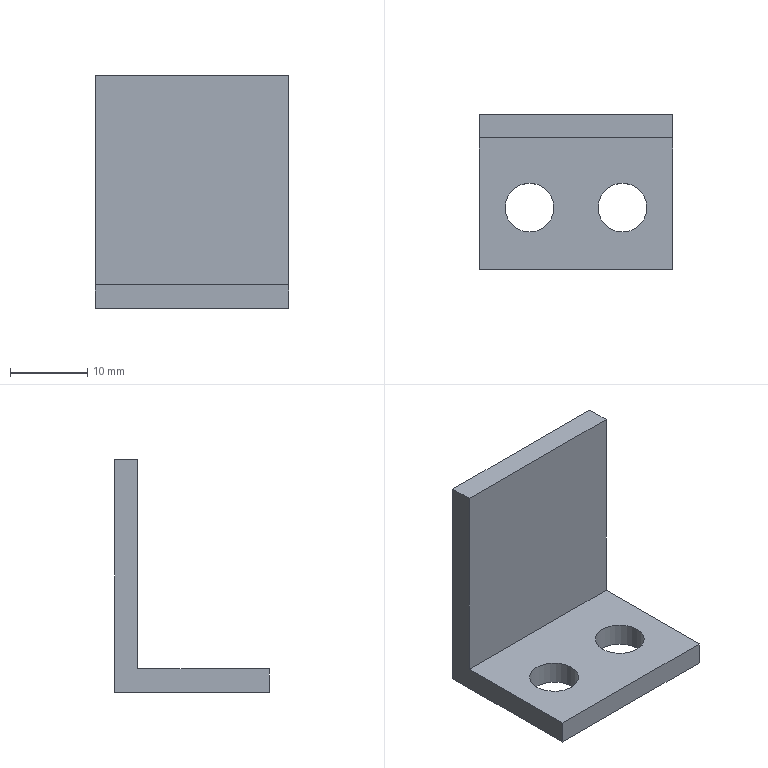Component | NX | SPRING_FIXING_PLATE | 1 solid | 10 faces | box 25 x 20 x 30 mm | volume 3338 mm3 | plane 8 | cylinder 2 | commonest cylinder face diameters 6.3 x2
STEP:
#1=CARTESIAN_POINT('',(0.,0.,0.));
#2=DIRECTION('',(0.,0.,1.));
#3=DIRECTION('',(1.,0.,0.));
#4=AXIS2_PLACEMENT_3D('',#1,#2,#3);
#5=CARTESIAN_POINT('',(-151.5,-8.,303.));
#6=VERTEX_POINT('',#5);
#7=CARTESIAN_POINT('',(-151.5,-25.,303.));
#8=VERTEX_POINT('',#7);
#9=CARTESIAN_POINT('',(-151.5,-5.,303.));
#10=DIRECTION('',(-0.,-1.,0.));
#11=VECTOR('',#10,1.);
#12=LINE('',#9,#11);
#13=CARTESIAN_POINT('',(-151.5,-5.,330.));
#14=DIRECTION('',(1.,-0.,0.));
#15=DIRECTION('',(0.,1.,0.));
#16=AXIS2_PLACEMENT_3D('',#13,#14,#15);
#17=PLANE('',#16);
#18=CARTESIAN_POINT('',(0.,-27.));
#19=DIRECTION('',(-1.,0.));
#20=VECTOR('',#19,1.);
#21=LINE('',#18,#20);
#22=(GEOMETRIC_REPRESENTATION_CONTEXT(2)PARAMETRIC_REPRESENTATION_CONTEXT()REPRESENTATION_CONTEXT('',''));
#23=DEFINITIONAL_REPRESENTATION('',(#21),#22);
#24=PCURVE('',#17,#23);
#25=CARTESIAN_POINT('',(-139.,-5.,303.));
#26=DIRECTION('',(0.,0.,1.));
#27=DIRECTION('',(1.,0.,0.));
#28=AXIS2_PLACEMENT_3D('',#25,#26,#27);
#29=PLANE('',#28);
#30=CARTESIAN_POINT('',(-12.5,0.));
#31=DIRECTION('',(-0.,-1.));
#32=VECTOR('',#31,1.);
#33=LINE('',#30,#32);
#34=(GEOMETRIC_REPRESENTATION_CONTEXT(2)PARAMETRIC_REPRESENTATION_CONTEXT()REPRESENTATION_CONTEXT('',''));
#35=DEFINITIONAL_REPRESENTATION('',(#33),#34);
#36=PCURVE('',#29,#35);
#37=SURFACE_CURVE('',#12,(#24,#36),.PCURVE_S1.);
#38=EDGE_CURVE('',#6,#8,#37,.T.);
#39=ORIENTED_EDGE('',*,*,#38,.F.);
#40=CARTESIAN_POINT('',(-151.5,-8.,330.));
#41=VERTEX_POINT('',#40);
#42=CARTESIAN_POINT('',(-151.5,-8.,330.));
#43=DIRECTION('',(0.,0.,-1.));
#44=VECTOR('',#43,1.);
#45=LINE('',#42,#44);
#46=CARTESIAN_POINT('',(-3.,0.));
#47=DIRECTION('',(0.,-1.));
#48=VECTOR('',#47,1.);
#49=LINE('',#46,#48);
#50=(GEOMETRIC_REPRESENTATION_CONTEXT(2)PARAMETRIC_REPRESENTATION_CONTEXT()REPRESENTATION_CONTEXT('',''));
#51=DEFINITIONAL_REPRESENTATION('',(#49),#50);
#52=PCURVE('',#17,#51);
#53=CARTESIAN_POINT('',(-126.5,-8.,330.));
#54=DIRECTION('',(0.,-1.,0.));
#55=DIRECTION('',(0.,0.,-1.));
#56=AXIS2_PLACEMENT_3D('',#53,#54,#55);
#57=PLANE('',#56);
#58=CARTESIAN_POINT('',(0.,-25.));
#59=DIRECTION('',(1.,0.));
#60=VECTOR('',#59,1.);
#61=LINE('',#58,#60);
#62=(GEOMETRIC_REPRESENTATION_CONTEXT(2)PARAMETRIC_REPRESENTATION_CONTEXT()REPRESENTATION_CONTEXT('',''));
#63=DEFINITIONAL_REPRESENTATION('',(#61),#62);
#64=PCURVE('',#57,#63);
#65=SURFACE_CURVE('',#45,(#52,#64),.PCURVE_S1.);
#66=EDGE_CURVE('',#41,#6,#65,.T.);
#67=ORIENTED_EDGE('',*,*,#66,.F.);
#68=CARTESIAN_POINT('',(-151.5,-5.,330.));
#69=VERTEX_POINT('',#68);
#70=CARTESIAN_POINT('',(-151.5,-5.,330.));
#71=DIRECTION('',(-0.,-1.,0.));
#72=VECTOR('',#71,1.);
#73=LINE('',#70,#72);
#74=CARTESIAN_POINT('',(0.,0.));
#75=DIRECTION('',(-1.,0.));
#76=VECTOR('',#75,1.);
#77=LINE('',#74,#76);
#78=(GEOMETRIC_REPRESENTATION_CONTEXT(2)PARAMETRIC_REPRESENTATION_CONTEXT()REPRESENTATION_CONTEXT('',''));
#79=DEFINITIONAL_REPRESENTATION('',(#77),#78);
#80=PCURVE('',#17,#79);
#81=CARTESIAN_POINT('',(-139.,-5.,330.));
#82=DIRECTION('',(0.,0.,1.));
#83=DIRECTION('',(1.,0.,0.));
#84=AXIS2_PLACEMENT_3D('',#81,#82,#83);
#85=PLANE('',#84);
#86=CARTESIAN_POINT('',(-12.5,0.));
#87=DIRECTION('',(-0.,-1.));
#88=VECTOR('',#87,1.);
#89=LINE('',#86,#88);
#90=(GEOMETRIC_REPRESENTATION_CONTEXT(2)PARAMETRIC_REPRESENTATION_CONTEXT()REPRESENTATION_CONTEXT('',''));
#91=DEFINITIONAL_REPRESENTATION('',(#89),#90);
#92=PCURVE('',#85,#91);
#93=SURFACE_CURVE('',#73,(#80,#92),.PCURVE_S1.);
#94=EDGE_CURVE('',#69,#41,#93,.T.);
#95=ORIENTED_EDGE('',*,*,#94,.F.);
#96=CARTESIAN_POINT('',(-151.5,-5.,300.));
#97=VERTEX_POINT('',#96);
#98=CARTESIAN_POINT('',(-151.5,-5.,330.));
#99=DIRECTION('',(0.,0.,-1.));
#100=VECTOR('',#99,1.);
#101=LINE('',#98,#100);
#102=CARTESIAN_POINT('',(0.,0.));
#103=DIRECTION('',(0.,-1.));
#104=VECTOR('',#103,1.);
#105=LINE('',#102,#104);
#106=(GEOMETRIC_REPRESENTATION_CONTEXT(2)PARAMETRIC_REPRESENTATION_CONTEXT()REPRESENTATION_CONTEXT('',''));
#107=DEFINITIONAL_REPRESENTATION('',(#105),#106);
#108=PCURVE('',#17,#107);
#109=CARTESIAN_POINT('',(-126.5,-5.,330.));
#110=DIRECTION('',(0.,-1.,0.));
#111=DIRECTION('',(0.,0.,-1.));
#112=AXIS2_PLACEMENT_3D('',#109,#110,#111);
#113=PLANE('',#112);
#114=CARTESIAN_POINT('',(0.,-25.));
#115=DIRECTION('',(1.,0.));
#116=VECTOR('',#115,1.);
#117=LINE('',#114,#116);
#118=(GEOMETRIC_REPRESENTATION_CONTEXT(2)PARAMETRIC_REPRESENTATION_CONTEXT()REPRESENTATION_CONTEXT('',''));
#119=DEFINITIONAL_REPRESENTATION('',(#117),#118);
#120=PCURVE('',#113,#119);
#121=SURFACE_CURVE('',#101,(#108,#120),.PCURVE_S1.);
#122=EDGE_CURVE('',#69,#97,#121,.T.);
#123=ORIENTED_EDGE('',*,*,#122,.T.);
#124=CARTESIAN_POINT('',(-151.5,-25.,300.));
#125=VERTEX_POINT('',#124);
#126=CARTESIAN_POINT('',(-151.5,-5.,300.));
#127=DIRECTION('',(-0.,-1.,0.));
#128=VECTOR('',#127,1.);
#129=LINE('',#126,#128);
#130=CARTESIAN_POINT('',(0.,-30.));
#131=DIRECTION('',(-1.,0.));
#132=VECTOR('',#131,1.);
#133=LINE('',#130,#132);
#134=(GEOMETRIC_REPRESENTATION_CONTEXT(2)PARAMETRIC_REPRESENTATION_CONTEXT()REPRESENTATION_CONTEXT('',''));
#135=DEFINITIONAL_REPRESENTATION('',(#133),#134);
#136=PCURVE('',#17,#135);
#137=CARTESIAN_POINT('',(-139.,-5.,300.));
#138=DIRECTION('',(0.,0.,1.));
#139=DIRECTION('',(1.,0.,0.));
#140=AXIS2_PLACEMENT_3D('',#137,#138,#139);
#141=PLANE('',#140);
#142=CARTESIAN_POINT('',(-12.5,0.));
#143=DIRECTION('',(-0.,-1.));
#144=VECTOR('',#143,1.);
#145=LINE('',#142,#144);
#146=(GEOMETRIC_REPRESENTATION_CONTEXT(2)PARAMETRIC_REPRESENTATION_CONTEXT()REPRESENTATION_CONTEXT('',''));
#147=DEFINITIONAL_REPRESENTATION('',(#145),#146);
#148=PCURVE('',#141,#147);
#149=SURFACE_CURVE('',#129,(#136,#148),.PCURVE_S1.);
#150=EDGE_CURVE('',#97,#125,#149,.T.);
#151=ORIENTED_EDGE('',*,*,#150,.T.);
#152=CARTESIAN_POINT('',(-151.5,-25.,330.));
#153=DIRECTION('',(0.,0.,-1.));
#154=VECTOR('',#153,1.);
#155=LINE('',#152,#154);
#156=CARTESIAN_POINT('',(-20.,0.));
#157=DIRECTION('',(0.,-1.));
#158=VECTOR('',#157,1.);
#159=LINE('',#156,#158);
#160=(GEOMETRIC_REPRESENTATION_CONTEXT(2)PARAMETRIC_REPRESENTATION_CONTEXT()REPRESENTATION_CONTEXT('',''));
#161=DEFINITIONAL_REPRESENTATION('',(#159),#160);
#162=PCURVE('',#17,#161);
#163=CARTESIAN_POINT('',(-151.5,-25.,330.));
#164=DIRECTION('',(0.,1.,0.));
#165=DIRECTION('',(0.,0.,1.));
#166=AXIS2_PLACEMENT_3D('',#163,#164,#165);
#167=PLANE('',#166);
#168=CARTESIAN_POINT('',(0.,0.));
#169=DIRECTION('',(-1.,0.));
#170=VECTOR('',#169,1.);
#171=LINE('',#168,#170);
#172=(GEOMETRIC_REPRESENTATION_CONTEXT(2)PARAMETRIC_REPRESENTATION_CONTEXT()REPRESENTATION_CONTEXT('',''));
#173=DEFINITIONAL_REPRESENTATION('',(#171),#172);
#174=PCURVE('',#167,#173);
#175=SURFACE_CURVE('',#155,(#162,#174),.PCURVE_S1.);
#176=EDGE_CURVE('',#8,#125,#175,.T.);
#177=ORIENTED_EDGE('',*,*,#176,.F.);
#178=EDGE_LOOP('',(#39,#67,#95,#123,#151,#177));
#179=FACE_BOUND('',#178,.T.);
#180=ADVANCED_FACE('',(#179),#17,.F.);
#181=CARTESIAN_POINT('',(-126.5,-25.,303.));
#182=VERTEX_POINT('',#181);
#183=CARTESIAN_POINT('',(-151.5,-25.,303.));
#184=DIRECTION('',(1.,0.,0.));
#185=VECTOR('',#184,1.);
#186=LINE('',#183,#185);
#187=CARTESIAN_POINT('',(-27.,0.));
#188=DIRECTION('',(0.,1.));
#189=VECTOR('',#188,1.);
#190=LINE('',#187,#189);
#191=(GEOMETRIC_REPRESENTATION_CONTEXT(2)PARAMETRIC_REPRESENTATION_CONTEXT()REPRESENTATION_CONTEXT('',''));
#192=DEFINITIONAL_REPRESENTATION('',(#190),#191);
#193=PCURVE('',#167,#192);
#194=CARTESIAN_POINT('',(-12.5,-20.));
#195=DIRECTION('',(1.,0.));
#196=VECTOR('',#195,1.);
#197=LINE('',#194,#196);
#198=(GEOMETRIC_REPRESENTATION_CONTEXT(2)PARAMETRIC_REPRESENTATION_CONTEXT()REPRESENTATION_CONTEXT('',''));
#199=DEFINITIONAL_REPRESENTATION('',(#197),#198);
#200=PCURVE('',#29,#199);
#201=SURFACE_CURVE('',#186,(#193,#200),.PCURVE_S1.);
#202=EDGE_CURVE('',#8,#182,#201,.T.);
#203=ORIENTED_EDGE('',*,*,#202,.F.);
#204=ORIENTED_EDGE('',*,*,#176,.T.);
#205=CARTESIAN_POINT('',(-126.5,-25.,300.));
#206=VERTEX_POINT('',#205);
#207=CARTESIAN_POINT('',(-151.5,-25.,300.));
#208=DIRECTION('',(1.,0.,0.));
#209=VECTOR('',#208,1.);
#210=LINE('',#207,#209);
#211=CARTESIAN_POINT('',(-30.,0.));
#212=DIRECTION('',(0.,1.));
#213=VECTOR('',#212,1.);
#214=LINE('',#211,#213);
#215=(GEOMETRIC_REPRESENTATION_CONTEXT(2)PARAMETRIC_REPRESENTATION_CONTEXT()REPRESENTATION_CONTEXT('',''));
#216=DEFINITIONAL_REPRESENTATION('',(#214),#215);
#217=PCURVE('',#167,#216);
#218=CARTESIAN_POINT('',(-12.5,-20.));
#219=DIRECTION('',(1.,0.));
#220=VECTOR('',#219,1.);
#221=LINE('',#218,#220);
#222=(GEOMETRIC_REPRESENTATION_CONTEXT(2)PARAMETRIC_REPRESENTATION_CONTEXT()REPRESENTATION_CONTEXT('',''));
#223=DEFINITIONAL_REPRESENTATION('',(#221),#222);
#224=PCURVE('',#141,#223);
#225=SURFACE_CURVE('',#210,(#217,#224),.PCURVE_S1.);
#226=EDGE_CURVE('',#125,#206,#225,.T.);
#227=ORIENTED_EDGE('',*,*,#226,.T.);
#228=CARTESIAN_POINT('',(-126.5,-25.,330.));
#229=DIRECTION('',(0.,0.,-1.));
#230=VECTOR('',#229,1.);
#231=LINE('',#228,#230);
#232=CARTESIAN_POINT('',(0.,25.));
#233=DIRECTION('',(-1.,0.));
#234=VECTOR('',#233,1.);
#235=LINE('',#232,#234);
#236=(GEOMETRIC_REPRESENTATION_CONTEXT(2)PARAMETRIC_REPRESENTATION_CONTEXT()REPRESENTATION_CONTEXT('',''));
#237=DEFINITIONAL_REPRESENTATION('',(#235),#236);
#238=PCURVE('',#167,#237);
#239=CARTESIAN_POINT('',(-126.5,-25.,330.));
#240=DIRECTION('',(-1.,-0.,0.));
#241=DIRECTION('',(0.,-1.,0.));
#242=AXIS2_PLACEMENT_3D('',#239,#240,#241);
#243=PLANE('',#242);
#244=CARTESIAN_POINT('',(0.,0.));
#245=DIRECTION('',(0.,-1.));
#246=VECTOR('',#245,1.);
#247=LINE('',#244,#246);
#248=(GEOMETRIC_REPRESENTATION_CONTEXT(2)PARAMETRIC_REPRESENTATION_CONTEXT()REPRESENTATION_CONTEXT('',''));
#249=DEFINITIONAL_REPRESENTATION('',(#247),#248);
#250=PCURVE('',#243,#249);
#251=SURFACE_CURVE('',#231,(#238,#250),.PCURVE_S1.);
#252=EDGE_CURVE('',#182,#206,#251,.T.);
#253=ORIENTED_EDGE('',*,*,#252,.F.);
#254=EDGE_LOOP('',(#203,#204,#227,#253));
#255=FACE_BOUND('',#254,.T.);
#256=ADVANCED_FACE('',(#255),#167,.F.);
#257=CARTESIAN_POINT('',(-126.5,-8.,303.));
#258=VERTEX_POINT('',#257);
#259=CARTESIAN_POINT('',(-126.5,-25.,303.));
#260=DIRECTION('',(-0.,1.,0.));
#261=VECTOR('',#260,1.);
#262=LINE('',#259,#261);
#263=CARTESIAN_POINT('',(0.,-27.));
#264=DIRECTION('',(-1.,0.));
#265=VECTOR('',#264,1.);
#266=LINE('',#263,#265);
#267=(GEOMETRIC_REPRESENTATION_CONTEXT(2)PARAMETRIC_REPRESENTATION_CONTEXT()REPRESENTATION_CONTEXT('',''));
#268=DEFINITIONAL_REPRESENTATION('',(#266),#267);
#269=PCURVE('',#243,#268);
#270=CARTESIAN_POINT('',(12.5,-20.));
#271=DIRECTION('',(-0.,1.));
#272=VECTOR('',#271,1.);
#273=LINE('',#270,#272);
#274=(GEOMETRIC_REPRESENTATION_CONTEXT(2)PARAMETRIC_REPRESENTATION_CONTEXT()REPRESENTATION_CONTEXT('',''));
#275=DEFINITIONAL_REPRESENTATION('',(#273),#274);
#276=PCURVE('',#29,#275);
#277=SURFACE_CURVE('',#262,(#269,#276),.PCURVE_S1.);
#278=EDGE_CURVE('',#182,#258,#277,.T.);
#279=ORIENTED_EDGE('',*,*,#278,.F.);
#280=ORIENTED_EDGE('',*,*,#252,.T.);
#281=CARTESIAN_POINT('',(-126.5,-5.,300.));
#282=VERTEX_POINT('',#281);
#283=CARTESIAN_POINT('',(-126.5,-25.,300.));
#284=DIRECTION('',(-0.,1.,0.));
#285=VECTOR('',#284,1.);
#286=LINE('',#283,#285);
#287=CARTESIAN_POINT('',(0.,-30.));
#288=DIRECTION('',(-1.,0.));
#289=VECTOR('',#288,1.);
#290=LINE('',#287,#289);
#291=(GEOMETRIC_REPRESENTATION_CONTEXT(2)PARAMETRIC_REPRESENTATION_CONTEXT()REPRESENTATION_CONTEXT('',''));
#292=DEFINITIONAL_REPRESENTATION('',(#290),#291);
#293=PCURVE('',#243,#292);
#294=CARTESIAN_POINT('',(12.5,-20.));
#295=DIRECTION('',(-0.,1.));
#296=VECTOR('',#295,1.);
#297=LINE('',#294,#296);
#298=(GEOMETRIC_REPRESENTATION_CONTEXT(2)PARAMETRIC_REPRESENTATION_CONTEXT()REPRESENTATION_CONTEXT('',''));
#299=DEFINITIONAL_REPRESENTATION('',(#297),#298);
#300=PCURVE('',#141,#299);
#301=SURFACE_CURVE('',#286,(#293,#300),.PCURVE_S1.);
#302=EDGE_CURVE('',#206,#282,#301,.T.);
#303=ORIENTED_EDGE('',*,*,#302,.T.);
#304=CARTESIAN_POINT('',(-126.5,-5.,330.));
#305=VERTEX_POINT('',#304);
#306=CARTESIAN_POINT('',(-126.5,-5.,330.));
#307=DIRECTION('',(0.,0.,-1.));
#308=VECTOR('',#307,1.);
#309=LINE('',#306,#308);
#310=CARTESIAN_POINT('',(-20.,0.));
#311=DIRECTION('',(0.,-1.));
#312=VECTOR('',#311,1.);
#313=LINE('',#310,#312);
#314=(GEOMETRIC_REPRESENTATION_CONTEXT(2)PARAMETRIC_REPRESENTATION_CONTEXT()REPRESENTATION_CONTEXT('',''));
#315=DEFINITIONAL_REPRESENTATION('',(#313),#314);
#316=PCURVE('',#243,#315);
#317=CARTESIAN_POINT('',(0.,0.));
#318=DIRECTION('',(1.,0.));
#319=VECTOR('',#318,1.);
#320=LINE('',#317,#319);
#321=(GEOMETRIC_REPRESENTATION_CONTEXT(2)PARAMETRIC_REPRESENTATION_CONTEXT()REPRESENTATION_CONTEXT('',''));
#322=DEFINITIONAL_REPRESENTATION('',(#320),#321);
#323=PCURVE('',#113,#322);
#324=SURFACE_CURVE('',#309,(#316,#323),.PCURVE_S1.);
#325=EDGE_CURVE('',#305,#282,#324,.T.);
#326=ORIENTED_EDGE('',*,*,#325,.F.);
#327=CARTESIAN_POINT('',(-126.5,-8.,330.));
#328=VERTEX_POINT('',#327);
#329=CARTESIAN_POINT('',(-126.5,-25.,330.));
#330=DIRECTION('',(-0.,1.,0.));
#331=VECTOR('',#330,1.);
#332=LINE('',#329,#331);
#333=CARTESIAN_POINT('',(0.,0.));
#334=DIRECTION('',(-1.,0.));
#335=VECTOR('',#334,1.);
#336=LINE('',#333,#335);
#337=(GEOMETRIC_REPRESENTATION_CONTEXT(2)PARAMETRIC_REPRESENTATION_CONTEXT()REPRESENTATION_CONTEXT('',''));
#338=DEFINITIONAL_REPRESENTATION('',(#336),#337);
#339=PCURVE('',#243,#338);
#340=CARTESIAN_POINT('',(12.5,-20.));
#341=DIRECTION('',(-0.,1.));
#342=VECTOR('',#341,1.);
#343=LINE('',#340,#342);
#344=(GEOMETRIC_REPRESENTATION_CONTEXT(2)PARAMETRIC_REPRESENTATION_CONTEXT()REPRESENTATION_CONTEXT('',''));
#345=DEFINITIONAL_REPRESENTATION('',(#343),#344);
#346=PCURVE('',#85,#345);
#347=SURFACE_CURVE('',#332,(#339,#346),.PCURVE_S1.);
#348=EDGE_CURVE('',#328,#305,#347,.T.);
#349=ORIENTED_EDGE('',*,*,#348,.F.);
#350=CARTESIAN_POINT('',(-126.5,-8.,330.));
#351=DIRECTION('',(0.,0.,-1.));
#352=VECTOR('',#351,1.);
#353=LINE('',#350,#352);
#354=CARTESIAN_POINT('',(-17.,0.));
#355=DIRECTION('',(0.,-1.));
#356=VECTOR('',#355,1.);
#357=LINE('',#354,#356);
#358=(GEOMETRIC_REPRESENTATION_CONTEXT(2)PARAMETRIC_REPRESENTATION_CONTEXT()REPRESENTATION_CONTEXT('',''));
#359=DEFINITIONAL_REPRESENTATION('',(#357),#358);
#360=PCURVE('',#243,#359);
#361=CARTESIAN_POINT('',(0.,0.));
#362=DIRECTION('',(1.,0.));
#363=VECTOR('',#362,1.);
#364=LINE('',#361,#363);
#365=(GEOMETRIC_REPRESENTATION_CONTEXT(2)PARAMETRIC_REPRESENTATION_CONTEXT()REPRESENTATION_CONTEXT('',''));
#366=DEFINITIONAL_REPRESENTATION('',(#364),#365);
#367=PCURVE('',#57,#366);
#368=SURFACE_CURVE('',#353,(#360,#367),.PCURVE_S1.);
#369=EDGE_CURVE('',#328,#258,#368,.T.);
#370=ORIENTED_EDGE('',*,*,#369,.T.);
#371=EDGE_LOOP('',(#279,#280,#303,#326,#349,#370));
#372=FACE_BOUND('',#371,.T.);
#373=ADVANCED_FACE('',(#372),#243,.F.);
#374=CARTESIAN_POINT('',(-126.5,-5.,300.));
#375=DIRECTION('',(-1.,0.,0.));
#376=VECTOR('',#375,1.);
#377=LINE('',#374,#376);
#378=CARTESIAN_POINT('',(30.,0.));
#379=DIRECTION('',(0.,-1.));
#380=VECTOR('',#379,1.);
#381=LINE('',#378,#380);
#382=(GEOMETRIC_REPRESENTATION_CONTEXT(2)PARAMETRIC_REPRESENTATION_CONTEXT()REPRESENTATION_CONTEXT('',''));
#383=DEFINITIONAL_REPRESENTATION('',(#381),#382);
#384=PCURVE('',#113,#383);
#385=CARTESIAN_POINT('',(12.5,0.));
#386=DIRECTION('',(-1.,0.));
#387=VECTOR('',#386,1.);
#388=LINE('',#385,#387);
#389=(GEOMETRIC_REPRESENTATION_CONTEXT(2)PARAMETRIC_REPRESENTATION_CONTEXT()REPRESENTATION_CONTEXT('',''));
#390=DEFINITIONAL_REPRESENTATION('',(#388),#389);
#391=PCURVE('',#141,#390);
#392=SURFACE_CURVE('',#377,(#384,#391),.PCURVE_S1.);
#393=EDGE_CURVE('',#282,#97,#392,.T.);
#394=ORIENTED_EDGE('',*,*,#393,.T.);
#395=ORIENTED_EDGE('',*,*,#122,.F.);
#396=CARTESIAN_POINT('',(-126.5,-5.,330.));
#397=DIRECTION('',(-1.,0.,0.));
#398=VECTOR('',#397,1.);
#399=LINE('',#396,#398);
#400=CARTESIAN_POINT('',(0.,0.));
#401=DIRECTION('',(0.,-1.));
#402=VECTOR('',#401,1.);
#403=LINE('',#400,#402);
#404=(GEOMETRIC_REPRESENTATION_CONTEXT(2)PARAMETRIC_REPRESENTATION_CONTEXT()REPRESENTATION_CONTEXT('',''));
#405=DEFINITIONAL_REPRESENTATION('',(#403),#404);
#406=PCURVE('',#113,#405);
#407=CARTESIAN_POINT('',(12.5,0.));
#408=DIRECTION('',(-1.,0.));
#409=VECTOR('',#408,1.);
#410=LINE('',#407,#409);
#411=(GEOMETRIC_REPRESENTATION_CONTEXT(2)PARAMETRIC_REPRESENTATION_CONTEXT()REPRESENTATION_CONTEXT('',''));
#412=DEFINITIONAL_REPRESENTATION('',(#410),#411);
#413=PCURVE('',#85,#412);
#414=SURFACE_CURVE('',#399,(#406,#413),.PCURVE_S1.);
#415=EDGE_CURVE('',#305,#69,#414,.T.);
#416=ORIENTED_EDGE('',*,*,#415,.F.);
#417=ORIENTED_EDGE('',*,*,#325,.T.);
#418=EDGE_LOOP('',(#394,#395,#416,#417));
#419=FACE_BOUND('',#418,.T.);
#420=ADVANCED_FACE('',(#419),#113,.F.);
#421=CARTESIAN_POINT('',(-126.5,-8.,330.));
#422=DIRECTION('',(-1.,0.,0.));
#423=VECTOR('',#422,1.);
#424=LINE('',#421,#423);
#425=CARTESIAN_POINT('',(12.5,-3.));
#426=DIRECTION('',(-1.,0.));
#427=VECTOR('',#426,1.);
#428=LINE('',#425,#427);
#429=(GEOMETRIC_REPRESENTATION_CONTEXT(2)PARAMETRIC_REPRESENTATION_CONTEXT()REPRESENTATION_CONTEXT('',''));
#430=DEFINITIONAL_REPRESENTATION('',(#428),#429);
#431=PCURVE('',#85,#430);
#432=CARTESIAN_POINT('',(0.,0.));
#433=DIRECTION('',(0.,-1.));
#434=VECTOR('',#433,1.);
#435=LINE('',#432,#434);
#436=(GEOMETRIC_REPRESENTATION_CONTEXT(2)PARAMETRIC_REPRESENTATION_CONTEXT()REPRESENTATION_CONTEXT('',''));
#437=DEFINITIONAL_REPRESENTATION('',(#435),#436);
#438=PCURVE('',#57,#437);
#439=SURFACE_CURVE('',#424,(#431,#438),.PCURVE_S1.);
#440=EDGE_CURVE('',#328,#41,#439,.T.);
#441=ORIENTED_EDGE('',*,*,#440,.F.);
#442=ORIENTED_EDGE('',*,*,#348,.T.);
#443=ORIENTED_EDGE('',*,*,#415,.T.);
#444=ORIENTED_EDGE('',*,*,#94,.T.);
#445=EDGE_LOOP('',(#441,#442,#443,#444));
#446=FACE_BOUND('',#445,.T.);
#447=ADVANCED_FACE('',(#446),#85,.T.);
#448=CARTESIAN_POINT('',(-129.85,-17.,300.));
#449=VERTEX_POINT('',#448);
#450=CARTESIAN_POINT('',(-136.15,-17.,300.));
#451=VERTEX_POINT('',#450);
#452=CARTESIAN_POINT('',(-133.,-17.,300.));
#453=DIRECTION('',(0.,0.,1.));
#454=DIRECTION('',(1.,0.,0.));
#455=AXIS2_PLACEMENT_3D('',#452,#453,#454);
#456=CIRCLE('',#455,3.15);
#457=CARTESIAN_POINT('',(6.,-12.));
#458=DIRECTION('',(1.,0.));
#459=AXIS2_PLACEMENT_2D('',#457,#458);
#460=CIRCLE('',#459,3.15);
#461=(GEOMETRIC_REPRESENTATION_CONTEXT(2)PARAMETRIC_REPRESENTATION_CONTEXT()REPRESENTATION_CONTEXT('',''));
#462=DEFINITIONAL_REPRESENTATION('',(#460),#461);
#463=PCURVE('',#141,#462);
#464=CARTESIAN_POINT('',(-133.,-17.,303.));
#465=DIRECTION('',(0.,0.,-1.));
#466=DIRECTION('',(-1.,0.,0.));
#467=AXIS2_PLACEMENT_3D('',#464,#465,#466);
#468=CYLINDRICAL_SURFACE('',#467,3.15);
#469=CARTESIAN_POINT('',(3.142,3.));
#470=DIRECTION('',(-1.,0.));
#471=VECTOR('',#470,1.);
#472=LINE('',#469,#471);
#473=(GEOMETRIC_REPRESENTATION_CONTEXT(2)PARAMETRIC_REPRESENTATION_CONTEXT()REPRESENTATION_CONTEXT('',''));
#474=DEFINITIONAL_REPRESENTATION('',(#472),#473);
#475=PCURVE('',#468,#474);
#476=SURFACE_CURVE('',#456,(#463,#475),.PCURVE_S1.);
#477=EDGE_CURVE('',#449,#451,#476,.T.);
#478=ORIENTED_EDGE('',*,*,#477,.T.);
#479=CARTESIAN_POINT('',(-133.,-17.,300.));
#480=DIRECTION('',(0.,0.,1.));
#481=DIRECTION('',(1.,0.,0.));
#482=AXIS2_PLACEMENT_3D('',#479,#480,#481);
#483=CIRCLE('',#482,3.15);
#484=CARTESIAN_POINT('',(6.,-12.));
#485=DIRECTION('',(1.,0.));
#486=AXIS2_PLACEMENT_2D('',#484,#485);
#487=CIRCLE('',#486,3.15);
#488=(GEOMETRIC_REPRESENTATION_CONTEXT(2)PARAMETRIC_REPRESENTATION_CONTEXT()REPRESENTATION_CONTEXT('',''));
#489=DEFINITIONAL_REPRESENTATION('',(#487),#488);
#490=PCURVE('',#141,#489);
#491=CARTESIAN_POINT('',(9.425,3.));
#492=DIRECTION('',(-1.,0.));
#493=VECTOR('',#492,1.);
#494=LINE('',#491,#493);
#495=(GEOMETRIC_REPRESENTATION_CONTEXT(2)PARAMETRIC_REPRESENTATION_CONTEXT()REPRESENTATION_CONTEXT('',''));
#496=DEFINITIONAL_REPRESENTATION('',(#494),#495);
#497=PCURVE('',#468,#496);
#498=SURFACE_CURVE('',#483,(#490,#497),.PCURVE_S1.);
#499=EDGE_CURVE('',#451,#449,#498,.T.);
#500=ORIENTED_EDGE('',*,*,#499,.T.);
#501=EDGE_LOOP('',(#478,#500));
#502=FACE_BOUND('',#501,.T.);
#503=CARTESIAN_POINT('',(-141.85,-17.,300.));
#504=VERTEX_POINT('',#503);
#505=CARTESIAN_POINT('',(-148.15,-17.,300.));
#506=VERTEX_POINT('',#505);
#507=CARTESIAN_POINT('',(-145.,-17.,300.));
#508=DIRECTION('',(0.,0.,1.));
#509=DIRECTION('',(1.,0.,0.));
#510=AXIS2_PLACEMENT_3D('',#507,#508,#509);
#511=CIRCLE('',#510,3.15);
#512=CARTESIAN_POINT('',(-6.,-12.));
#513=DIRECTION('',(1.,0.));
#514=AXIS2_PLACEMENT_2D('',#512,#513);
#515=CIRCLE('',#514,3.15);
#516=(GEOMETRIC_REPRESENTATION_CONTEXT(2)PARAMETRIC_REPRESENTATION_CONTEXT()REPRESENTATION_CONTEXT('',''));
#517=DEFINITIONAL_REPRESENTATION('',(#515),#516);
#518=PCURVE('',#141,#517);
#519=CARTESIAN_POINT('',(-145.,-17.,303.));
#520=DIRECTION('',(0.,0.,-1.));
#521=DIRECTION('',(-1.,0.,0.));
#522=AXIS2_PLACEMENT_3D('',#519,#520,#521);
#523=CYLINDRICAL_SURFACE('',#522,3.15);
#524=CARTESIAN_POINT('',(3.142,3.));
#525=DIRECTION('',(-1.,0.));
#526=VECTOR('',#525,1.);
#527=LINE('',#524,#526);
#528=(GEOMETRIC_REPRESENTATION_CONTEXT(2)PARAMETRIC_REPRESENTATION_CONTEXT()REPRESENTATION_CONTEXT('',''));
#529=DEFINITIONAL_REPRESENTATION('',(#527),#528);
#530=PCURVE('',#523,#529);
#531=SURFACE_CURVE('',#511,(#518,#530),.PCURVE_S1.);
#532=EDGE_CURVE('',#504,#506,#531,.T.);
#533=ORIENTED_EDGE('',*,*,#532,.T.);
#534=CARTESIAN_POINT('',(-145.,-17.,300.));
#535=DIRECTION('',(0.,0.,1.));
#536=DIRECTION('',(1.,0.,0.));
#537=AXIS2_PLACEMENT_3D('',#534,#535,#536);
#538=CIRCLE('',#537,3.15);
#539=CARTESIAN_POINT('',(-6.,-12.));
#540=DIRECTION('',(1.,0.));
#541=AXIS2_PLACEMENT_2D('',#539,#540);
#542=CIRCLE('',#541,3.15);
#543=(GEOMETRIC_REPRESENTATION_CONTEXT(2)PARAMETRIC_REPRESENTATION_CONTEXT()REPRESENTATION_CONTEXT('',''));
#544=DEFINITIONAL_REPRESENTATION('',(#542),#543);
#545=PCURVE('',#141,#544);
#546=CARTESIAN_POINT('',(9.425,3.));
#547=DIRECTION('',(-1.,0.));
#548=VECTOR('',#547,1.);
#549=LINE('',#546,#548);
#550=(GEOMETRIC_REPRESENTATION_CONTEXT(2)PARAMETRIC_REPRESENTATION_CONTEXT()REPRESENTATION_CONTEXT('',''));
#551=DEFINITIONAL_REPRESENTATION('',(#549),#550);
#552=PCURVE('',#523,#551);
#553=SURFACE_CURVE('',#538,(#545,#552),.PCURVE_S1.);
#554=EDGE_CURVE('',#506,#504,#553,.T.);
#555=ORIENTED_EDGE('',*,*,#554,.T.);
#556=EDGE_LOOP('',(#533,#555));
#557=FACE_BOUND('',#556,.T.);
#558=ORIENTED_EDGE('',*,*,#150,.F.);
#559=ORIENTED_EDGE('',*,*,#393,.F.);
#560=ORIENTED_EDGE('',*,*,#302,.F.);
#561=ORIENTED_EDGE('',*,*,#226,.F.);
#562=EDGE_LOOP('',(#558,#559,#560,#561));
#563=FACE_BOUND('',#562,.T.);
#564=ADVANCED_FACE('',(#502,#557,#563),#141,.F.);
#565=CARTESIAN_POINT('',(-126.5,-8.,303.));
#566=DIRECTION('',(-1.,0.,0.));
#567=VECTOR('',#566,1.);
#568=LINE('',#565,#567);
#569=CARTESIAN_POINT('',(27.,0.));
#570=DIRECTION('',(0.,-1.));
#571=VECTOR('',#570,1.);
#572=LINE('',#569,#571);
#573=(GEOMETRIC_REPRESENTATION_CONTEXT(2)PARAMETRIC_REPRESENTATION_CONTEXT()REPRESENTATION_CONTEXT('',''));
#574=DEFINITIONAL_REPRESENTATION('',(#572),#573);
#575=PCURVE('',#57,#574);
#576=CARTESIAN_POINT('',(12.5,-3.));
#577=DIRECTION('',(-1.,0.));
#578=VECTOR('',#577,1.);
#579=LINE('',#576,#578);
#580=(GEOMETRIC_REPRESENTATION_CONTEXT(2)PARAMETRIC_REPRESENTATION_CONTEXT()REPRESENTATION_CONTEXT('',''));
#581=DEFINITIONAL_REPRESENTATION('',(#579),#580);
#582=PCURVE('',#29,#581);
#583=SURFACE_CURVE('',#568,(#575,#582),.PCURVE_S1.);
#584=EDGE_CURVE('',#258,#6,#583,.T.);
#585=ORIENTED_EDGE('',*,*,#584,.F.);
#586=ORIENTED_EDGE('',*,*,#369,.F.);
#587=ORIENTED_EDGE('',*,*,#440,.T.);
#588=ORIENTED_EDGE('',*,*,#66,.T.);
#589=EDGE_LOOP('',(#585,#586,#587,#588));
#590=FACE_BOUND('',#589,.T.);
#591=ADVANCED_FACE('',(#590),#57,.T.);
#592=CARTESIAN_POINT('',(-136.15,-17.,303.));
#593=VERTEX_POINT('',#592);
#594=CARTESIAN_POINT('',(-133.,-17.,303.));
#595=DIRECTION('',(0.,0.,-1.));
#596=DIRECTION('',(-1.,0.,0.));
#597=AXIS2_PLACEMENT_3D('',#594,#595,#596);
#598=CIRCLE('',#597,3.15);
#599=CARTESIAN_POINT('',(2.85,-12.));
#600=CARTESIAN_POINT('',(2.85,-6.544));
#601=CARTESIAN_POINT('',(7.575,-9.272));
#602=CARTESIAN_POINT('',(12.3,-12.));
#603=CARTESIAN_POINT('',(7.575,-14.728));
#604=CARTESIAN_POINT('',(2.85,-17.456));
#605=CARTESIAN_POINT('',(2.85,-12.));
#606=(BOUNDED_CURVE()B_SPLINE_CURVE(2,(#599,#600,#601,#602,#603,#604,#605),.UNSPECIFIED.,.T.,.F.)B_SPLINE_CURVE_WITH_KNOTS((1,2,2,2,2,1),(-2.094,0.,2.094,4.189,6.283,8.378),.UNSPECIFIED.)CURVE()GEOMETRIC_REPRESENTATION_ITEM()RATIONAL_B_SPLINE_CURVE((1.,0.5,1.,0.5,1.,0.5,1.))REPRESENTATION_ITEM(''));
#607=(GEOMETRIC_REPRESENTATION_CONTEXT(2)PARAMETRIC_REPRESENTATION_CONTEXT()REPRESENTATION_CONTEXT('',''));
#608=DEFINITIONAL_REPRESENTATION('',(#606),#607);
#609=PCURVE('',#29,#608);
#610=CARTESIAN_POINT('',(0.,0.));
#611=DIRECTION('',(1.,0.));
#612=VECTOR('',#611,1.);
#613=LINE('',#610,#612);
#614=(GEOMETRIC_REPRESENTATION_CONTEXT(2)PARAMETRIC_REPRESENTATION_CONTEXT()REPRESENTATION_CONTEXT('',''));
#615=DEFINITIONAL_REPRESENTATION('',(#613),#614);
#616=PCURVE('',#468,#615);
#617=SURFACE_CURVE('',#598,(#609,#616),.PCURVE_S1.);
#618=EDGE_CURVE('',#593,#593,#617,.T.);
#619=ORIENTED_EDGE('',*,*,#618,.T.);
#620=EDGE_LOOP('',(#619));
#621=FACE_BOUND('',#620,.T.);
#622=CARTESIAN_POINT('',(-148.15,-17.,303.));
#623=VERTEX_POINT('',#622);
#624=CARTESIAN_POINT('',(-145.,-17.,303.));
#625=DIRECTION('',(0.,0.,-1.));
#626=DIRECTION('',(-1.,0.,0.));
#627=AXIS2_PLACEMENT_3D('',#624,#625,#626);
#628=CIRCLE('',#627,3.15);
#629=CARTESIAN_POINT('',(-9.15,-12.));
#630=CARTESIAN_POINT('',(-9.15,-6.544));
#631=CARTESIAN_POINT('',(-4.425,-9.272));
#632=CARTESIAN_POINT('',(0.3,-12.));
#633=CARTESIAN_POINT('',(-4.425,-14.728));
#634=CARTESIAN_POINT('',(-9.15,-17.456));
#635=CARTESIAN_POINT('',(-9.15,-12.));
#636=(BOUNDED_CURVE()B_SPLINE_CURVE(2,(#629,#630,#631,#632,#633,#634,#635),.UNSPECIFIED.,.T.,.F.)B_SPLINE_CURVE_WITH_KNOTS((1,2,2,2,2,1),(-2.094,0.,2.094,4.189,6.283,8.378),.UNSPECIFIED.)CURVE()GEOMETRIC_REPRESENTATION_ITEM()RATIONAL_B_SPLINE_CURVE((1.,0.5,1.,0.5,1.,0.5,1.))REPRESENTATION_ITEM(''));
#637=(GEOMETRIC_REPRESENTATION_CONTEXT(2)PARAMETRIC_REPRESENTATION_CONTEXT()REPRESENTATION_CONTEXT('',''));
#638=DEFINITIONAL_REPRESENTATION('',(#636),#637);
#639=PCURVE('',#29,#638);
#640=CARTESIAN_POINT('',(0.,0.));
#641=DIRECTION('',(1.,0.));
#642=VECTOR('',#641,1.);
#643=LINE('',#640,#642);
#644=(GEOMETRIC_REPRESENTATION_CONTEXT(2)PARAMETRIC_REPRESENTATION_CONTEXT()REPRESENTATION_CONTEXT('',''));
#645=DEFINITIONAL_REPRESENTATION('',(#643),#644);
#646=PCURVE('',#523,#645);
#647=SURFACE_CURVE('',#628,(#639,#646),.PCURVE_S1.);
#648=EDGE_CURVE('',#623,#623,#647,.T.);
#649=ORIENTED_EDGE('',*,*,#648,.T.);
#650=EDGE_LOOP('',(#649));
#651=FACE_BOUND('',#650,.T.);
#652=ORIENTED_EDGE('',*,*,#38,.T.);
#653=ORIENTED_EDGE('',*,*,#202,.T.);
#654=ORIENTED_EDGE('',*,*,#278,.T.);
#655=ORIENTED_EDGE('',*,*,#584,.T.);
#656=EDGE_LOOP('',(#652,#653,#654,#655));
#657=FACE_BOUND('',#656,.T.);
#658=ADVANCED_FACE('',(#621,#651,#657),#29,.T.);
#659=ORIENTED_EDGE('',*,*,#648,.T.);
#660=CARTESIAN_POINT('',(-148.15,-17.,303.));
#661=CARTESIAN_POINT('',(-148.15,-17.,300.));
#662=B_SPLINE_CURVE_WITH_KNOTS('',1,(#660,#661),.UNSPECIFIED.,.F.,.F.,(2,2),(0.,3.),.PIECEWISE_BEZIER_KNOTS.);
#663=CARTESIAN_POINT('',(6.283,0.));
#664=DIRECTION('',(0.,1.));
#665=VECTOR('',#664,1.);
#666=LINE('',#663,#665);
#667=(GEOMETRIC_REPRESENTATION_CONTEXT(2)PARAMETRIC_REPRESENTATION_CONTEXT()REPRESENTATION_CONTEXT('',''));
#668=DEFINITIONAL_REPRESENTATION('',(#666),#667);
#669=PCURVE('',#523,#668);
#670=CARTESIAN_POINT('',(0.,0.));
#671=DIRECTION('',(0.,1.));
#672=VECTOR('',#671,1.);
#673=LINE('',#670,#672);
#674=(GEOMETRIC_REPRESENTATION_CONTEXT(2)PARAMETRIC_REPRESENTATION_CONTEXT()REPRESENTATION_CONTEXT('',''));
#675=DEFINITIONAL_REPRESENTATION('',(#673),#674);
#676=PCURVE('',#523,#675);
#677=SEAM_CURVE('',#662,(#669,#676),.PCURVE_S1.);
#678=EDGE_CURVE('',#623,#506,#677,.T.);
#679=ORIENTED_EDGE('',*,*,#678,.T.);
#680=ORIENTED_EDGE('',*,*,#554,.T.);
#681=ORIENTED_EDGE('',*,*,#532,.T.);
#682=ORIENTED_EDGE('',*,*,#678,.F.);
#683=EDGE_LOOP('',(#659,#679,#680,#681,#682));
#684=FACE_BOUND('',#683,.F.);
#685=ADVANCED_FACE('',(#684),#523,.F.);
#686=ORIENTED_EDGE('',*,*,#618,.T.);
#687=CARTESIAN_POINT('',(-136.15,-17.,303.));
#688=CARTESIAN_POINT('',(-136.15,-17.,300.));
#689=B_SPLINE_CURVE_WITH_KNOTS('',1,(#687,#688),.UNSPECIFIED.,.F.,.F.,(2,2),(0.,3.),.PIECEWISE_BEZIER_KNOTS.);
#690=CARTESIAN_POINT('',(6.283,0.));
#691=DIRECTION('',(0.,1.));
#692=VECTOR('',#691,1.);
#693=LINE('',#690,#692);
#694=(GEOMETRIC_REPRESENTATION_CONTEXT(2)PARAMETRIC_REPRESENTATION_CONTEXT()REPRESENTATION_CONTEXT('',''));
#695=DEFINITIONAL_REPRESENTATION('',(#693),#694);
#696=PCURVE('',#468,#695);
#697=CARTESIAN_POINT('',(0.,0.));
#698=DIRECTION('',(0.,1.));
#699=VECTOR('',#698,1.);
#700=LINE('',#697,#699);
#701=(GEOMETRIC_REPRESENTATION_CONTEXT(2)PARAMETRIC_REPRESENTATION_CONTEXT()REPRESENTATION_CONTEXT('',''));
#702=DEFINITIONAL_REPRESENTATION('',(#700),#701);
#703=PCURVE('',#468,#702);
#704=SEAM_CURVE('',#689,(#696,#703),.PCURVE_S1.);
#705=EDGE_CURVE('',#593,#451,#704,.T.);
#706=ORIENTED_EDGE('',*,*,#705,.T.);
#707=ORIENTED_EDGE('',*,*,#499,.T.);
#708=ORIENTED_EDGE('',*,*,#477,.T.);
#709=ORIENTED_EDGE('',*,*,#705,.F.);
#710=EDGE_LOOP('',(#686,#706,#707,#708,#709));
#711=FACE_BOUND('',#710,.F.);
#712=ADVANCED_FACE('',(#711),#468,.F.);
#713=CLOSED_SHELL('',(#180,#256,#373,#420,#447,#564,#591,#658,#685,#712));
#714=MANIFOLD_SOLID_BREP('',#713);
#715=(LENGTH_UNIT()NAMED_UNIT(*)SI_UNIT(.MILLI.,.METRE.));
#716=UNCERTAINTY_MEASURE_WITH_UNIT(LENGTH_MEASURE(0.000002),#715,'','');
#717=(NAMED_UNIT(*)PLANE_ANGLE_UNIT()SI_UNIT($,.RADIAN.));
#718=(NAMED_UNIT(*)SI_UNIT($,.STERADIAN.)SOLID_ANGLE_UNIT());
#719=(GEOMETRIC_REPRESENTATION_CONTEXT(3)GLOBAL_UNCERTAINTY_ASSIGNED_CONTEXT((#716))GLOBAL_UNIT_ASSIGNED_CONTEXT((#715,#717,#718))REPRESENTATION_CONTEXT('',''));
#720=ADVANCED_BREP_SHAPE_REPRESENTATION('',(#4,#714),#719);